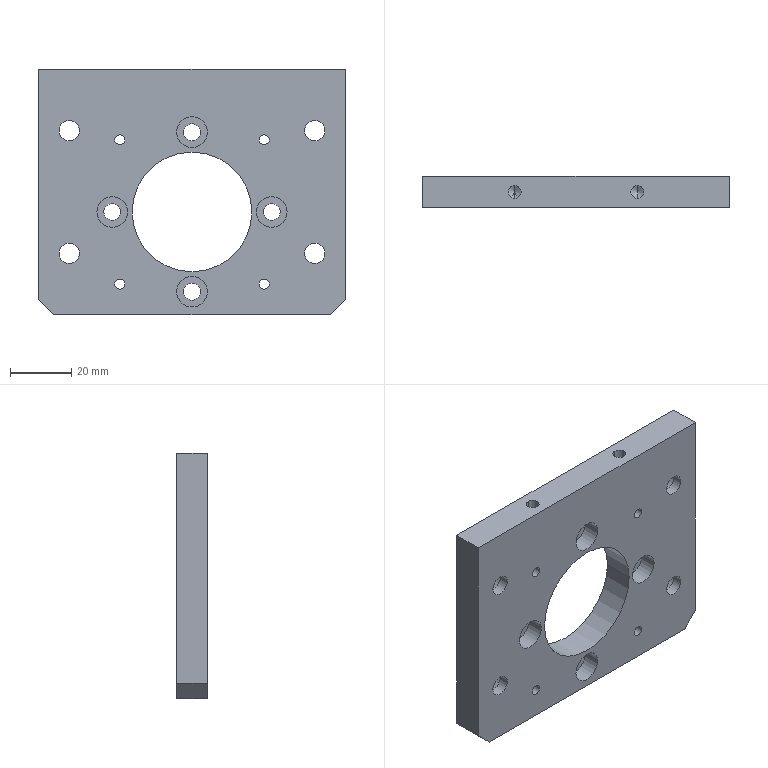Component | SolidWorks | 75-02-20StirringMotorConnectionPlateModified-1 | 1 solid | 66 faces | box 100 x 10 x 80 mm | volume 61885 mm3 | cylinder 46 | plane 16 | cone 4 | commonest cylinder face diameters 11 x8 6.6 x8 10 x8 5.5 x8 3.3 x8 4.2 x4 39 x2 | material A3 Steel
build123d program:
from build123d import *

# Parameters (mm, degrees)
SKETCH1_W                                          = 100
SKETCH1_H                                          = 80
BOSS_EXTRUDE1_DEPTH                                = 5
M4_TAPPED_HOLE1_D                                  = 3.3
M5_TAPPED_HOLE1_D                                  = 4.2
M5_TAPPED_HOLE1_DEPTH                              = 12.4
M5_TAPPED_HOLE1_TIP                                = 1.262
SKETCH10_R                                         = 19.5
CUT_EXTRUDE1_DEPTH                                 = 65.807
CHAMFER1_SIZE                                      = 5
HOLE_SIZE_ACCORDING_TO_TYPE_OF_HEXAGON_D           = 5.5
HOLE_SIZE_ACCORDING_TO_TYPE_OF_HEXAGON_CBORE_D     = 10
HOLE_SIZE_ACCORDING_TO_TYPE_OF_HEXAGON_CBORE_DEPTH = 5.7
CIRPATTERN1_COUNT                                  = 4
HOLE_SIZE_ACCORDING_TO_TYPE_OF_HEX_2_D             = 6.6
HOLE_SIZE_ACCORDING_TO_TYPE_OF_HEX_2_CBORE_D       = 11
HOLE_SIZE_ACCORDING_TO_TYPE_OF_HEX_2_CBORE_DEPTH   = 6.8


with BuildPart() as part:
    # Sketch1 → Boss-Extrude1 (new, symmetric)
    with BuildSketch(Plane.XY):
        Rectangle(SKETCH1_W, SKETCH1_H)
    extrude(amount=BOSS_EXTRUDE1_DEPTH, both=True)

    # M4 Tapped Hole1 (through all)
    with Locations(Plane(origin=(-23.5, 30, 5), x_dir=(1, 0, 0), z_dir=(0, 0, 1))):
        with Locations((0, 0), (0, -47), (47, 0), (47, -47)):
            Hole(M4_TAPPED_HOLE1_D / 2)

    # M5 Tapped Hole1
    with Locations(Plane(origin=(-20, -40, 0), x_dir=(0, 0, -1), z_dir=(0, -1, 0))):
        with Locations((0, 0), (0, 40)):
            Hole(M5_TAPPED_HOLE1_D / 2, depth=M5_TAPPED_HOLE1_DEPTH)
            with Locations((0, 0, -(M5_TAPPED_HOLE1_DEPTH + M5_TAPPED_HOLE1_TIP / 2))):  # 118° drill point
                Cone(0, M5_TAPPED_HOLE1_D / 2, M5_TAPPED_HOLE1_TIP, mode=Mode.SUBTRACT)

    # Sketch10 → Cut-Extrude1 (cut, through all)
    with BuildSketch(Plane.XY.offset(5)):
        with Locations((0, 6.5)):
            Circle(SKETCH10_R)
    extrude(amount=-CUT_EXTRUDE1_DEPTH, mode=Mode.SUBTRACT)

    # Chamfer1
    chamfer1_edges = [part.edges().sort_by_distance(p)[0] for p in [
        (-50, 40, 0),
        (50, 40, 0),
    ]]
    chamfer(chamfer1_edges, length=CHAMFER1_SIZE)

    # Hole Size _according to_ Type of Hexagon (through all)
    with Locations(Plane(origin=(0, 32.5, -5), x_dir=(-1, 0, 0), z_dir=(0, 0, -1))):
        with Locations((0, 0)):
            hole_size_according_to_type_of_hexagon = CounterBoreHole(HOLE_SIZE_ACCORDING_TO_TYPE_OF_HEXAGON_D / 2, HOLE_SIZE_ACCORDING_TO_TYPE_OF_HEXAGON_CBORE_D / 2, HOLE_SIZE_ACCORDING_TO_TYPE_OF_HEXAGON_CBORE_DEPTH)

    # CirPattern1: Hole Size _according to_ Type of Hexagon ×4 about axis
    cirpattern1_axis = Axis((0, 6.5, 0), (0, 0, 1))
    for i in range(1, CIRPATTERN1_COUNT):
        add(hole_size_according_to_type_of_hexagon.rotate(cirpattern1_axis, i * 360 / CIRPATTERN1_COUNT), mode=Mode.SUBTRACT)

    # Hole Size _according to_ Type of Hex 2 (through all)
    with Locations(Plane(origin=(-40, 20, 5), x_dir=(1, 0, 0), z_dir=(0, 0, 1))):
        with Locations((0, 0), (80, 0), (80, -40), (0, -40)):
            CounterBoreHole(HOLE_SIZE_ACCORDING_TO_TYPE_OF_HEX_2_D / 2, HOLE_SIZE_ACCORDING_TO_TYPE_OF_HEX_2_CBORE_D / 2, HOLE_SIZE_ACCORDING_TO_TYPE_OF_HEX_2_CBORE_DEPTH)


solid = part.part

# Placed as in the assembly
solid = solid.moved(Location((-17.8, 110.857, -37.25), (-90, 0, 0)))